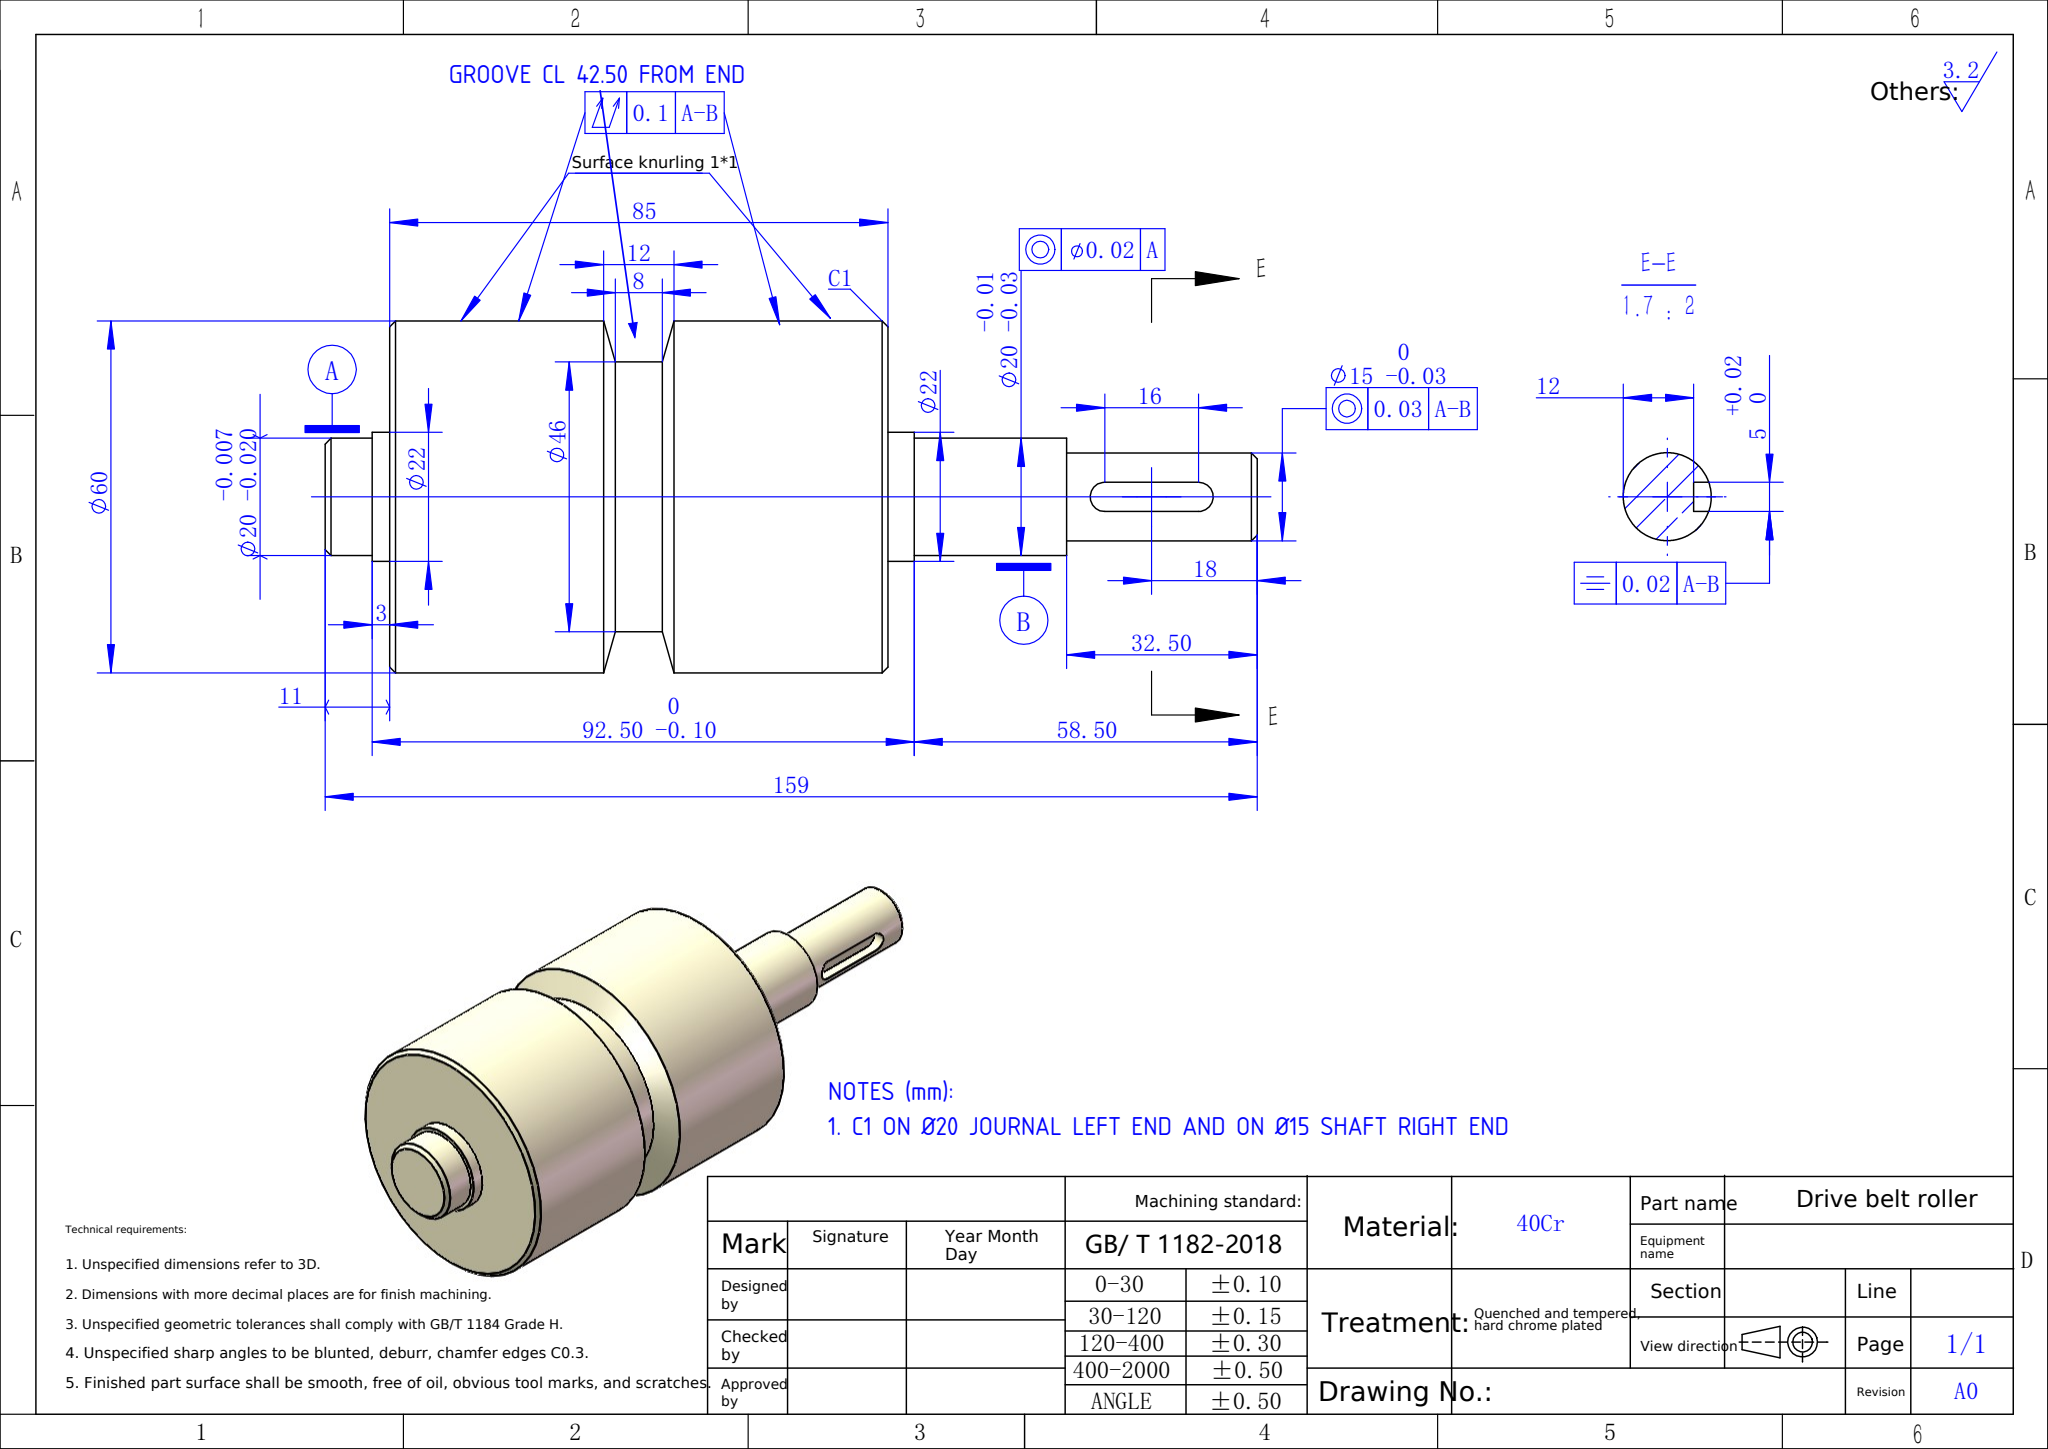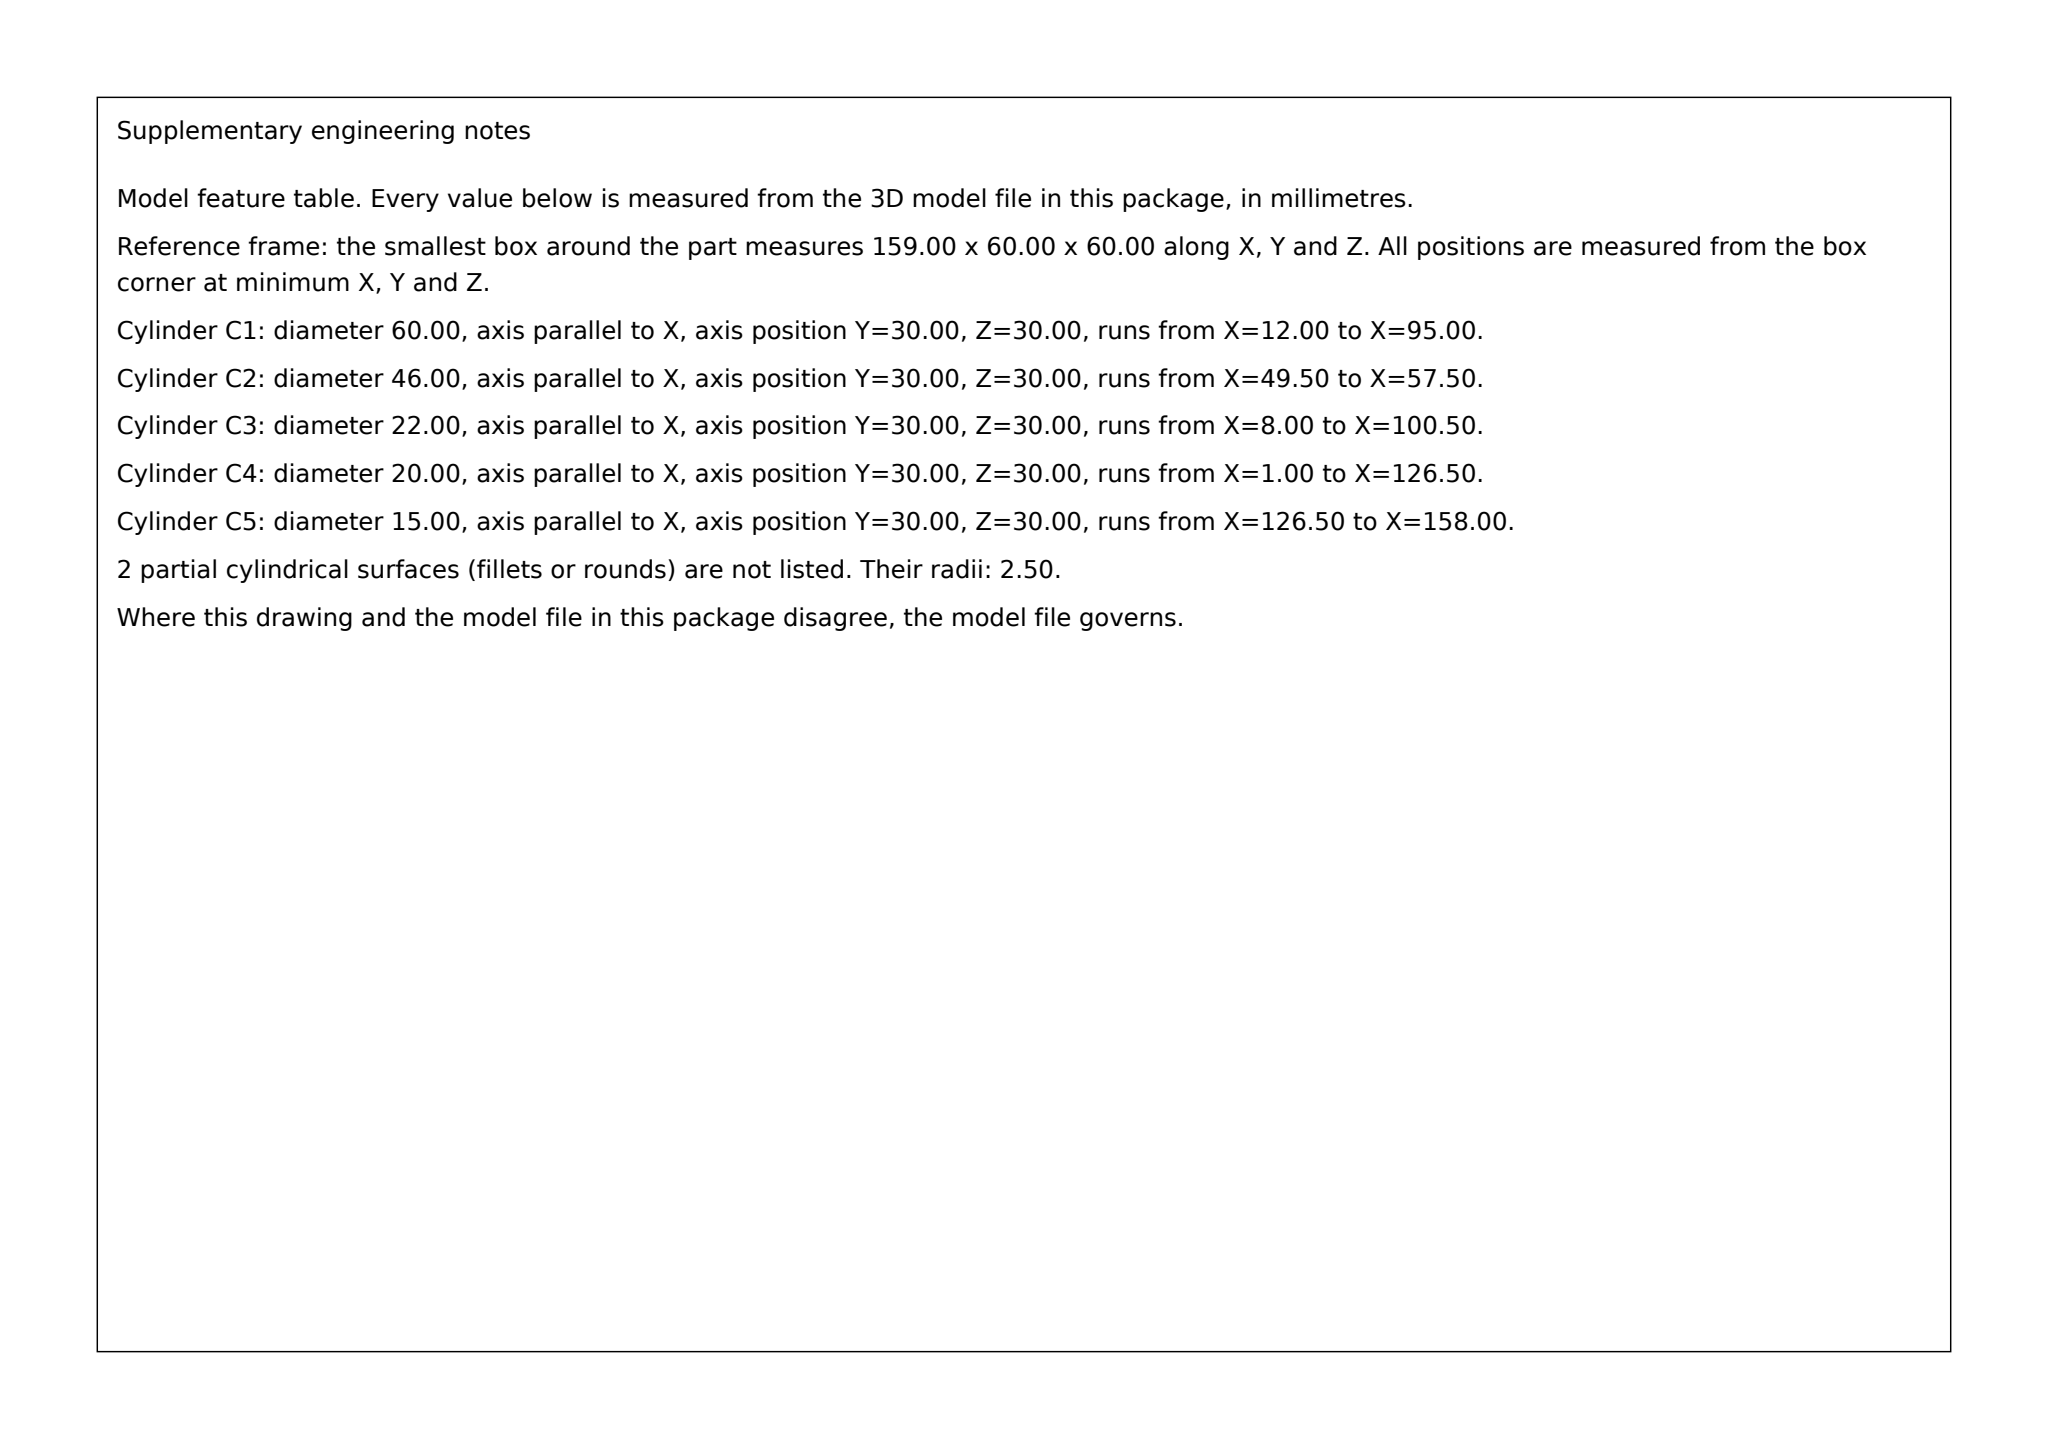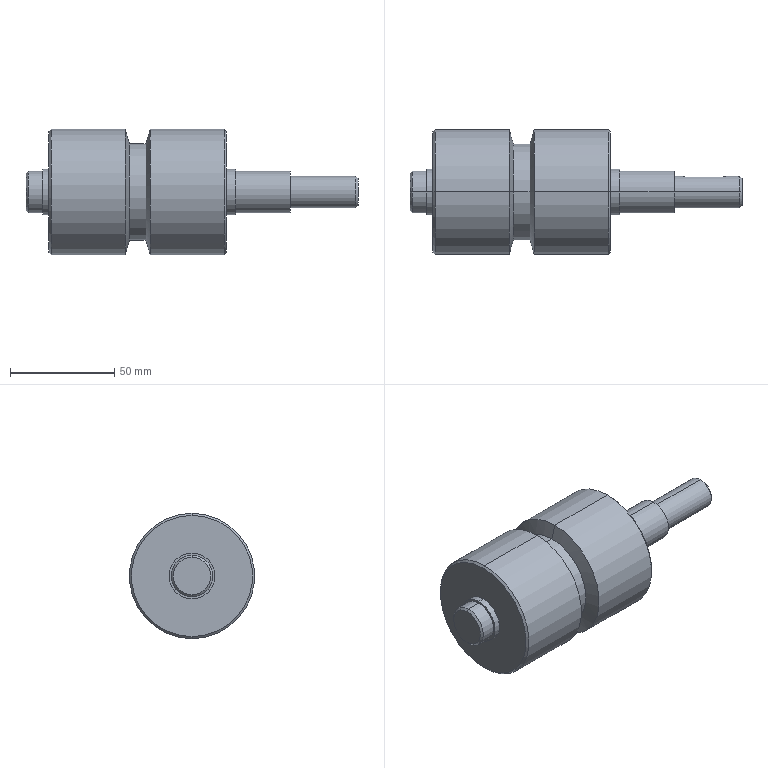Part | SolidWorks | mm | material 40Cr | 1 solid | 40 faces | box 159 x 60 x 60 mm | volume 247325 mm3 | cylinder 18 | cone 12 | plane 10 | commonest cylinder face diameters 20 x4 22 x4 60 x4 46 x2 15 x2 5 x2
Drawing notes:
Ø46 GROOVE CL 42.50 FROM EA Ø60 END FACE (CTR ON 85) | from the solid: Ø60 body x=11..96 (85 lg); Ø46 groove bottom x=49.5..57.5, OD opening x=47.5..59.5 -> CL x=53.5 = 42.5 from each Ø60 face
C1 ON Ø20 JOURNAL LEFT END AND ON Ø15 SHAFT RIGHT END | from the solid: 90° cones ref dia 18 at x=0 (Ø20->Ø18) and ref dia 15 at x=158..159 (Ø15->Ø13) = 1 mm x 45°